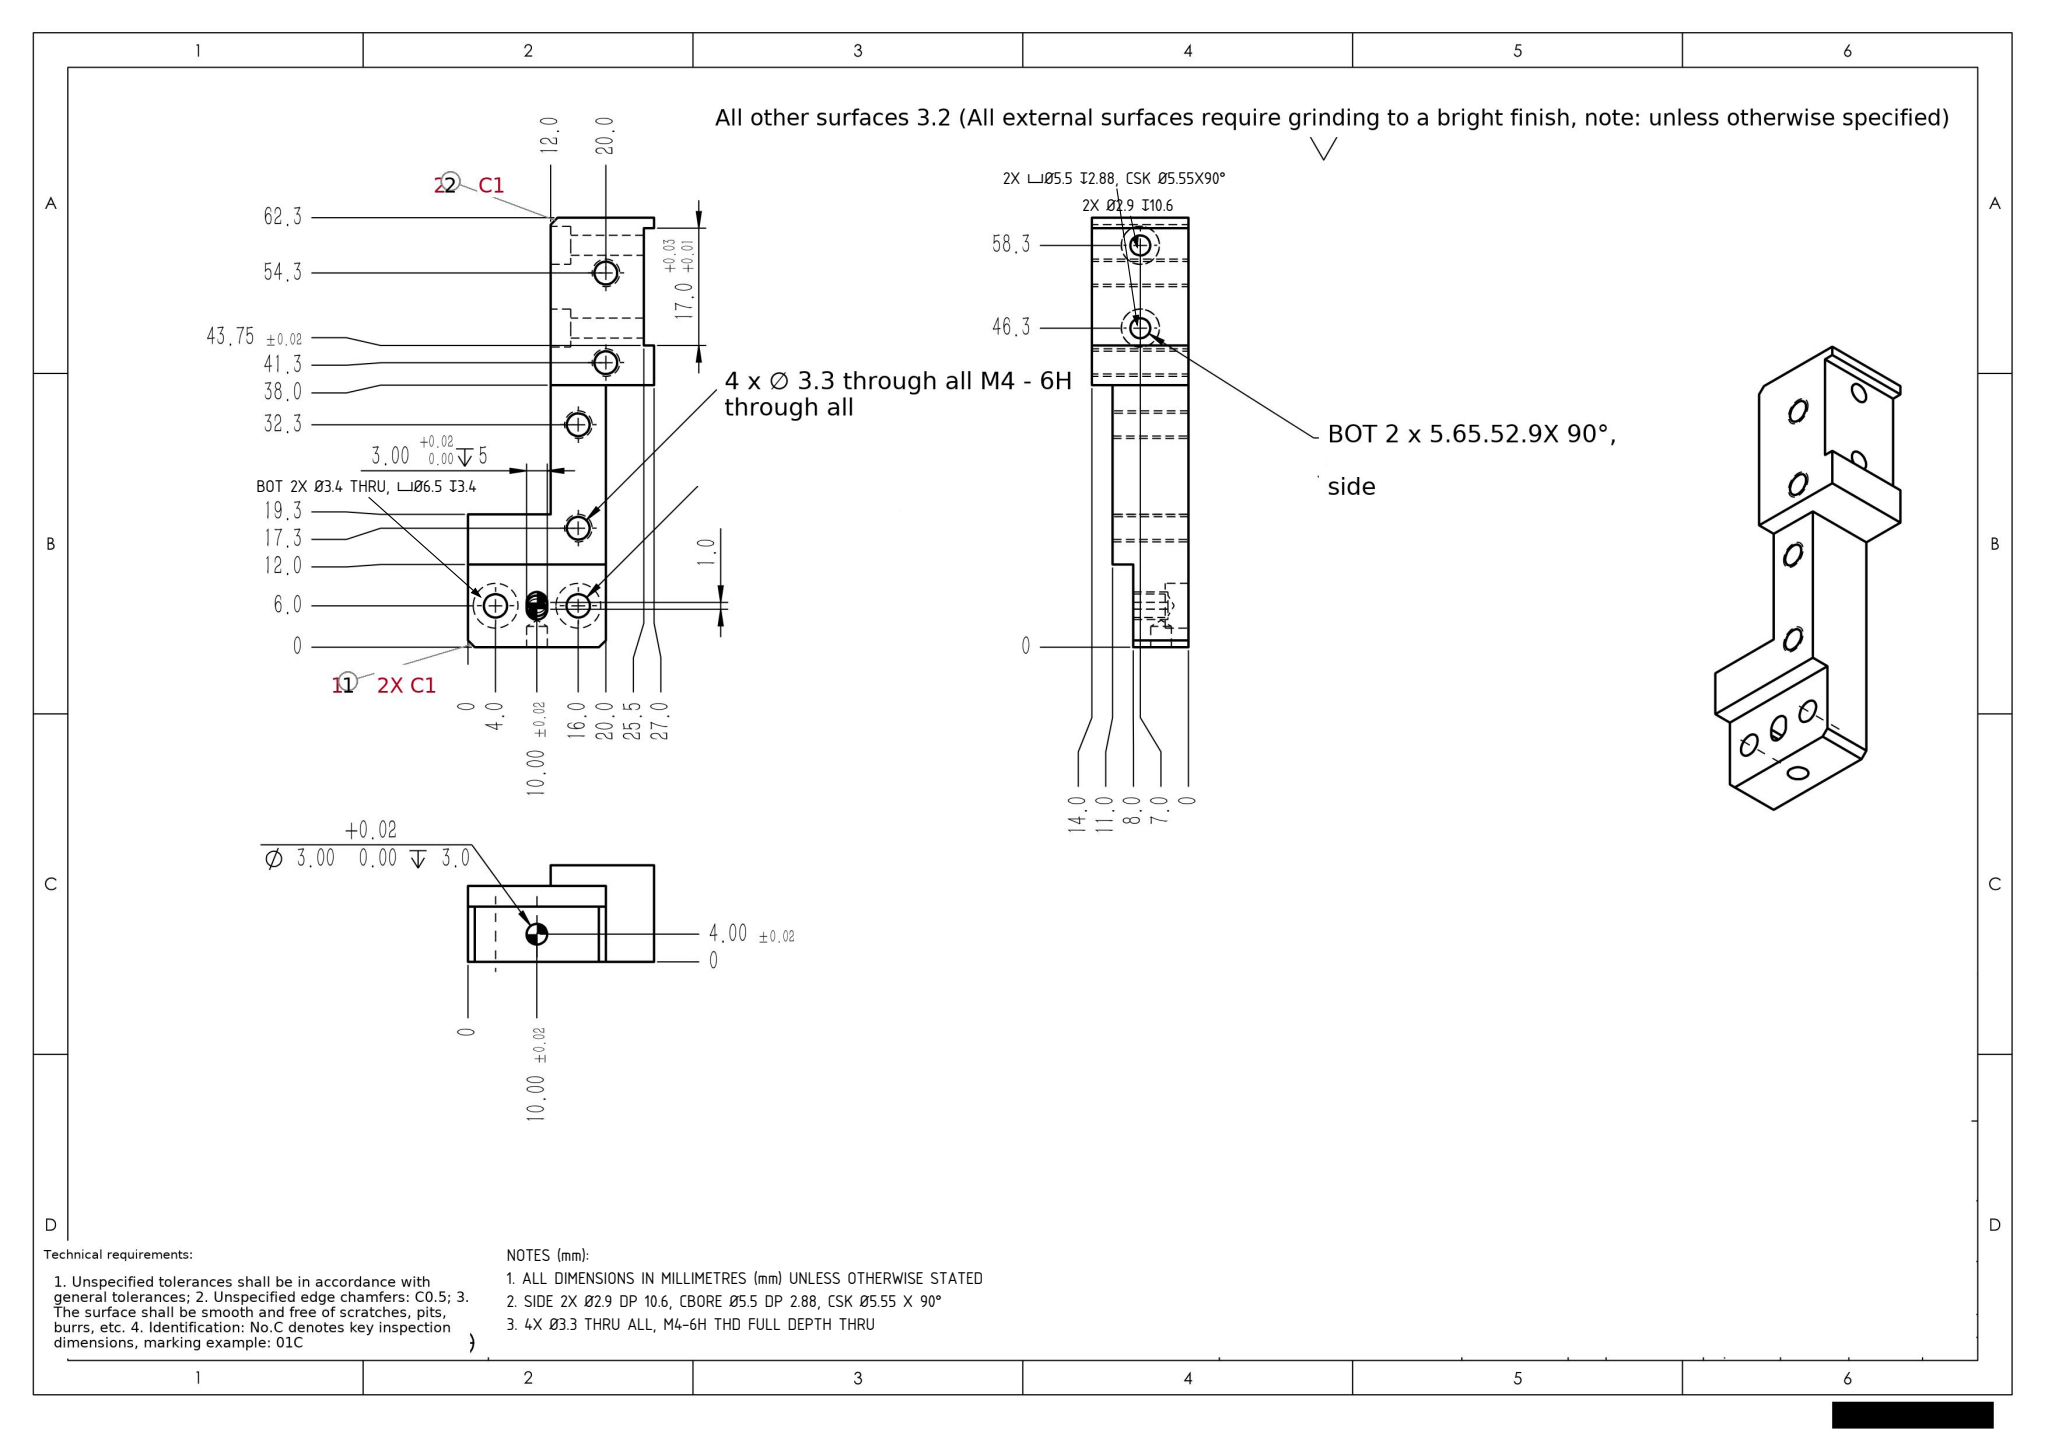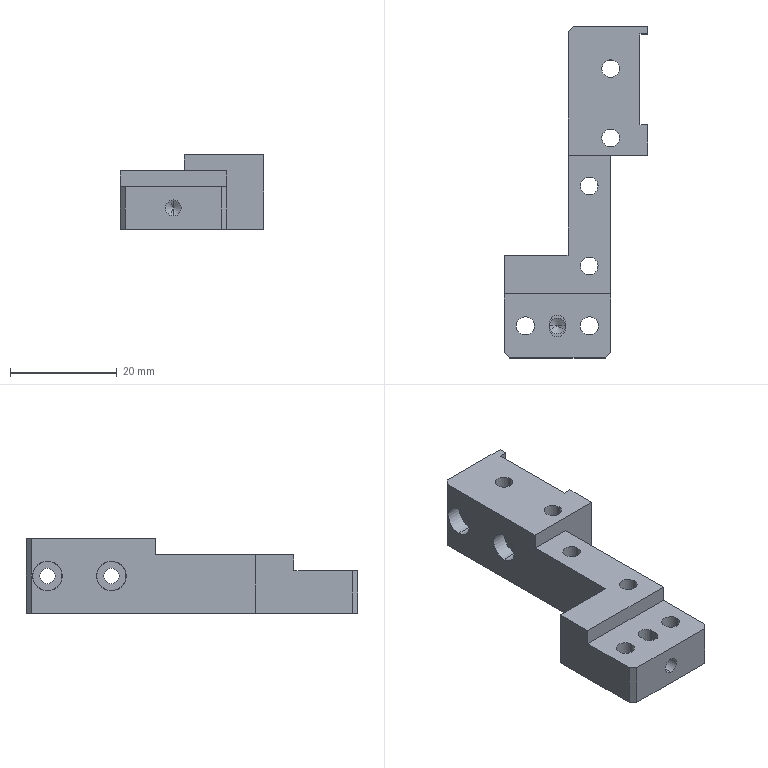Part | SolidWorks | mm | 1 solid | 64 faces | box 27 x 62.25 x 14 mm | volume 8795 mm3 | cylinder 28 | plane 28 | cone 8 | commonest cylinder face diameters 3.3 x8 3 x4 6.5 x4 3.4 x4 5.5 x4 2.9 x4
Drawing notes:
ALL DIMENSIONS IN MILLIMETRES (mm) UNLESS OTHERWISE STATED | from the solid: STEP model facts stated in mm; bbox_xyz 27.0 x 62.25 x 14.0 mm
BOT 2X Ø3.4 THRU, CBORE Ø6.5 DP 3.4 (AT X=4 & X=16, Y=6) | from the solid: cyl 3.4 z @ (4,6) & (16,6) len 4.6 thru; cyl 6.5 z @ same, len 3.4
SIDE 2X Ø2.9 DP 10.6 (AT Y=46.3 & 58.3, Z=7) | from the solid: cyl 2.9 axis x @ (y46.25,z7) & (y58.25,z7), len 10.6
SIDE 2X CBORE Ø5.5 DP 2.88, CSK Ø5.55 X 90° | from the solid: cyl 5.5 axis x len 2.88 @ y46.25/58.25 z7; cone 90° ref dia 5.55
SIDE 2X Ø2.9 DP 10.6, CBORE Ø5.5 DP 2.88, CSK Ø5.55 X 90° | from the solid: replaces merged 'BOT 2 x 5.65.52.9X 90' callout: 2.9x10.6, 5.5x2.88, 90° csk Ø5.55
4X Ø3.3 THRU ALL, M4-6H THD FULL DEPTH THRU | from the solid: cyl 3.3 len 11 @ (16,17.25)&(16,32.25); len 14 @ (20,41.25)&(20,54.25) = full wall
build123d program:
from build123d import *

# Parameters (mm, degrees)
SKETCH1_W                                       = 27
SKETCH1_H                                       = 62.25
BOSS_EXTRUDE1_DEPTH                             = 14
SKETCH8_W                                       = 6
SKETCH8_H                                       = 12
CUT_EXTRUDE7_DEPTH                              = 70.282
SKETCH9_W                                       = 1.5
SKETCH9_H                                       = 17
CUT_EXTRUDE8_DEPTH                              = 70.282
SKETCH10_W                                      = 7
SKETCH10_H                                      = 38
CUT_EXTRUDE9_DEPTH                              = 70.282
SKETCH11_W                                      = 12
SKETCH11_H                                      = 43
CUT_EXTRUDE10_DEPTH                             = 70.282
M2_5_HEX_SOCKET_HEAD_CAP_SCREW_CBORE1_AT_COUNT  = 2
M2_5_HEX_SOCKET_HEAD_CAP_SCREW_CBORE1_AT_PITCH  = 12
CHAMFER2_SIZE                                   = 1
M3_HEX_SOCKET_HEAD_CAP_SCREW_CBORE1_D           = 3.4
M3_HEX_SOCKET_HEAD_CAP_SCREW_CBORE1_CBORE_D     = 6.5
M3_HEX_SOCKET_HEAD_CAP_SCREW_CBORE1_CBORE_DEPTH = 3.4
CHAMFER1_SIZE                                   = 1
SKETCH16_W                                      = 3
SKETCH16_H                                      = 26
CUT_EXTRUDE11_DEPTH                             = 67.866
SIZE_MM_DOWEL_PIN_HOLE1_D                       = 3
SIZE_MM_DOWEL_PIN_HOLE1_DEPTH                   = 5
SIZE_MM_DOWEL_PIN_HOLE1_TIP                     = 0.9013
CUT_EXTRUDE12_DEPTH                             = 5
M4_TAPPED_HOLE1_D                               = 3.3
SIZE_MM_DOWEL_PIN_HOLE2_D                       = 3
SIZE_MM_DOWEL_PIN_HOLE2_DEPTH                   = 3
SIZE_MM_DOWEL_PIN_HOLE2_TIP                     = 0.9013


with BuildPart() as part:
    # Sketch1 → Boss-Extrude1 (new body)
    with BuildSketch(Plane.XY):
        with Locations((13.5, 31.125)):
            Rectangle(SKETCH1_W, SKETCH1_H)
    extrude(amount=BOSS_EXTRUDE1_DEPTH)

    # Sketch8 → Cut-Extrude7 (cut, through all)
    with BuildSketch(Plane.ZY):
        with Locations((11, 6)):
            Rectangle(SKETCH8_W, SKETCH8_H)
    extrude(amount=-CUT_EXTRUDE7_DEPTH, mode=Mode.SUBTRACT)

    # Sketch9 → Cut-Extrude8 (cut, through all)
    with BuildSketch(Plane(origin=(0, 0, 0), x_dir=(-1, 0, 0), z_dir=(0, 0, -1))):
        with Locations((-26.25, 52.25)):
            Rectangle(SKETCH9_W, SKETCH9_H)
    extrude(amount=-CUT_EXTRUDE8_DEPTH, mode=Mode.SUBTRACT)

    # Sketch10 → Cut-Extrude9 (cut, through all)
    with BuildSketch(Plane(origin=(0, 0, 0), x_dir=(-1, 0, 0), z_dir=(0, 0, -1))):
        with Locations((-23.5, 19)):
            Rectangle(SKETCH10_W, SKETCH10_H)
    extrude(amount=-CUT_EXTRUDE9_DEPTH, mode=Mode.SUBTRACT)

    # Sketch11 → Cut-Extrude10 (cut, through all)
    with BuildSketch(Plane(origin=(0, 0, 0), x_dir=(-1, 0, 0), z_dir=(0, 0, -1))):
        with Locations((-6, 40.75)):
            Rectangle(SKETCH11_W, SKETCH11_H)
    extrude(amount=-CUT_EXTRUDE10_DEPTH, mode=Mode.SUBTRACT)

    # Sketch13 → M2.5 Hex Socket Head Cap Screw CBORE1 (revolve, cut)
    with BuildSketch(Plane(origin=(12, 46.25, 7), x_dir=(0, 0, 1), z_dir=(0, 1, 0))):
        Polygon((0, 0), (0, 15), (1.45, 15), (1.45, 2.9), (2.75, 2.9), (2.75, 0.025), (2.775, 0), align=None)
    m2_5_hex_socket_head_cap_screw_cbore1 = revolve(axis=Axis((5.65, 46.25, 7), (1, 0, 0)), mode=Mode.SUBTRACT)

    # M2.5 Hex Socket Head Cap Screw CBORE1 at: M2.5 Hex Socket Head Cap Screw CBORE1 ×2
    with Locations(*[(0, i * M2_5_HEX_SOCKET_HEAD_CAP_SCREW_CBORE1_AT_PITCH, 0) for i in range(1, M2_5_HEX_SOCKET_HEAD_CAP_SCREW_CBORE1_AT_COUNT)]):
        add(m2_5_hex_socket_head_cap_screw_cbore1, mode=Mode.SUBTRACT)

    # Chamfer2
    chamfer2_edges = [part.edges().sort_by_distance(p)[0] for p in [
        (12, 62.25, 7),
    ]]
    chamfer(chamfer2_edges, length=CHAMFER2_SIZE)

    # M3 Hex Socket Head Cap Screw CBORE1 (through all)
    with Locations(Plane(origin=(0, 0, 0), x_dir=(-1, 0, 0), z_dir=(0, 0, -1))):
        with Locations((-4, 6), (-16, 6)):
            CounterBoreHole(M3_HEX_SOCKET_HEAD_CAP_SCREW_CBORE1_D / 2, M3_HEX_SOCKET_HEAD_CAP_SCREW_CBORE1_CBORE_D / 2, M3_HEX_SOCKET_HEAD_CAP_SCREW_CBORE1_CBORE_DEPTH)

    # Chamfer1
    chamfer1_edges = [part.edges().sort_by_distance(p)[0] for p in [
        (0, 0, 4),
        (20, 0, 4),
    ]]
    chamfer(chamfer1_edges, length=CHAMFER1_SIZE)

    # Sketch16 → Cut-Extrude11 (cut, through all)
    with BuildSketch(Plane(origin=(20, 0, 0), x_dir=(0, 0, -1), z_dir=(1, 0, 0))):
        with Locations((-12.5, 25)):
            Rectangle(SKETCH16_W, SKETCH16_H)
    extrude(amount=-CUT_EXTRUDE11_DEPTH, mode=Mode.SUBTRACT)

    # Size mm Dowel Pin Hole1
    with Locations(Plane(origin=(0, 0, 8), x_dir=(-1, 0, 0), z_dir=(0, 0, 1))):
        with Locations((-10, -6)):
            Hole(SIZE_MM_DOWEL_PIN_HOLE1_D / 2, depth=SIZE_MM_DOWEL_PIN_HOLE1_DEPTH)
            with Locations((0, 0, -(SIZE_MM_DOWEL_PIN_HOLE1_DEPTH + SIZE_MM_DOWEL_PIN_HOLE1_TIP / 2))):  # 118° drill point
                Cone(0, SIZE_MM_DOWEL_PIN_HOLE1_D / 2, SIZE_MM_DOWEL_PIN_HOLE1_TIP, mode=Mode.SUBTRACT)

    # Sketch19 → Cut-Extrude12 (cut)
    with BuildSketch(Plane(origin=(0, 0, 8), x_dir=(-1, 0, 0), z_dir=(0, 0, -1))):
        with BuildLine():
            Line((-11.5, 5.5), (-11.5, 6.5))
            ThreePointArc((-11.5, 6.5), (-10, 8), (-8.5, 6.5))
            Line((-8.5, 6.5), (-8.5, 5.5))
            ThreePointArc((-8.5, 5.5), (-10, 4), (-11.5, 5.5))
        make_face()
    extrude(amount=CUT_EXTRUDE12_DEPTH, mode=Mode.SUBTRACT)

    # M4 Tapped Hole1 (through all)
    with Locations(Plane.XY.offset(14)):
        with Locations((16, 32.25), (16, 17.25), (20, 54.25), (20, 41.25)):
            Hole(M4_TAPPED_HOLE1_D / 2)

    # Size mm Dowel Pin Hole2
    with Locations(Plane(origin=(0, 0, 0), x_dir=(-1, 0, 0), z_dir=(0, -1, 0))):
        with Locations((-10, -4)):
            Hole(SIZE_MM_DOWEL_PIN_HOLE2_D / 2, depth=SIZE_MM_DOWEL_PIN_HOLE2_DEPTH)
            with Locations((0, 0, -(SIZE_MM_DOWEL_PIN_HOLE2_DEPTH + SIZE_MM_DOWEL_PIN_HOLE2_TIP / 2))):  # 118° drill point
                Cone(0, SIZE_MM_DOWEL_PIN_HOLE2_D / 2, SIZE_MM_DOWEL_PIN_HOLE2_TIP, mode=Mode.SUBTRACT)


solid = part.part